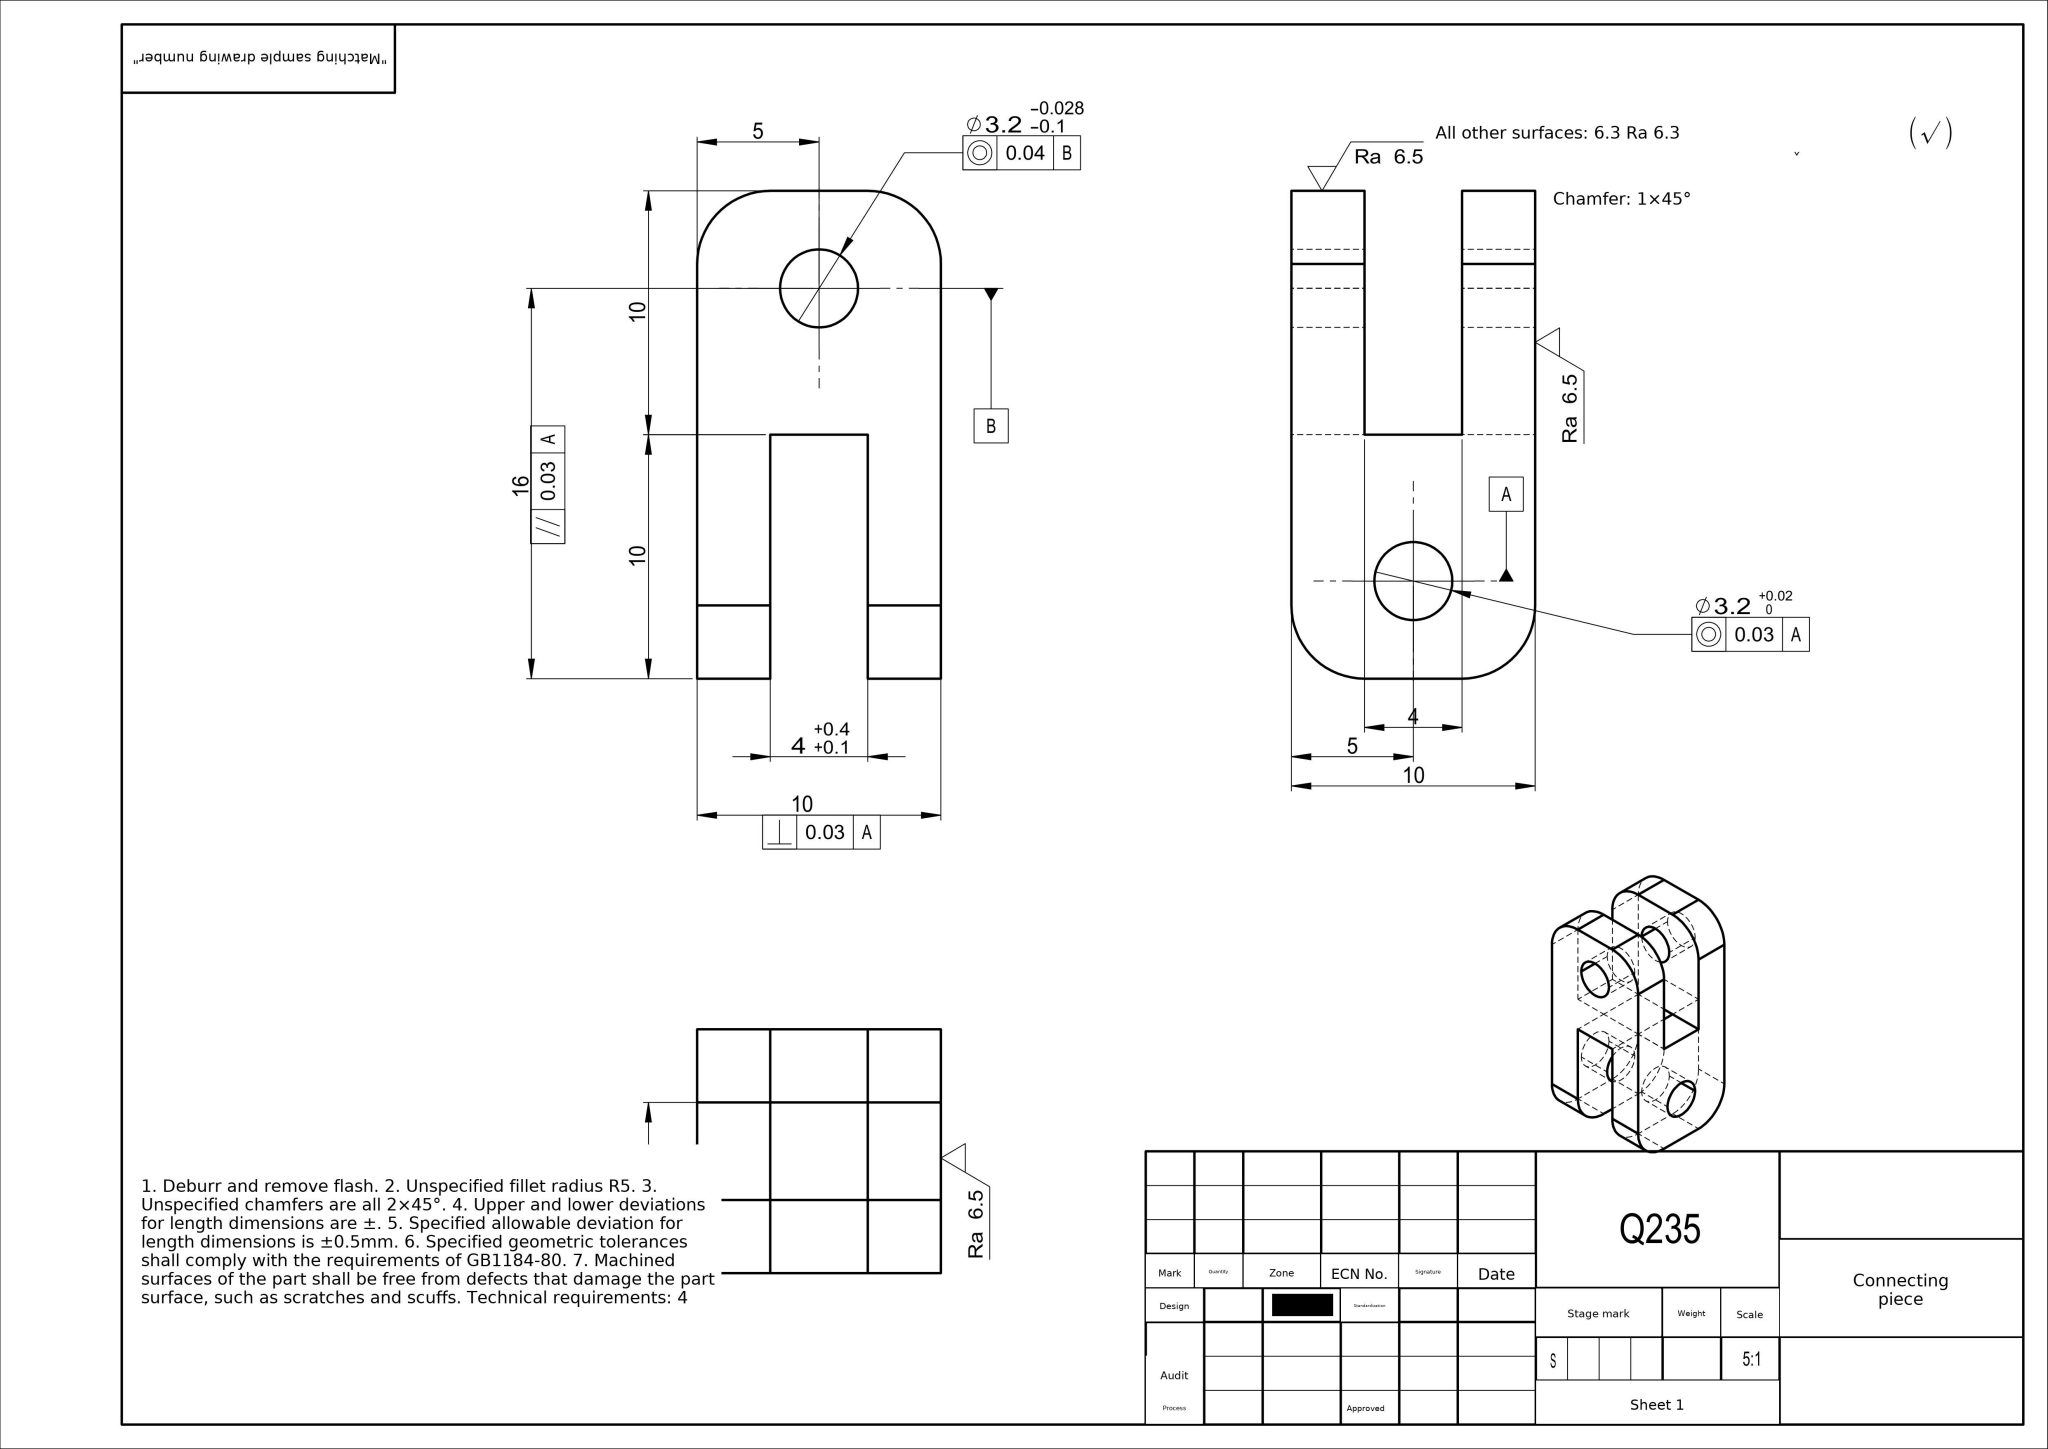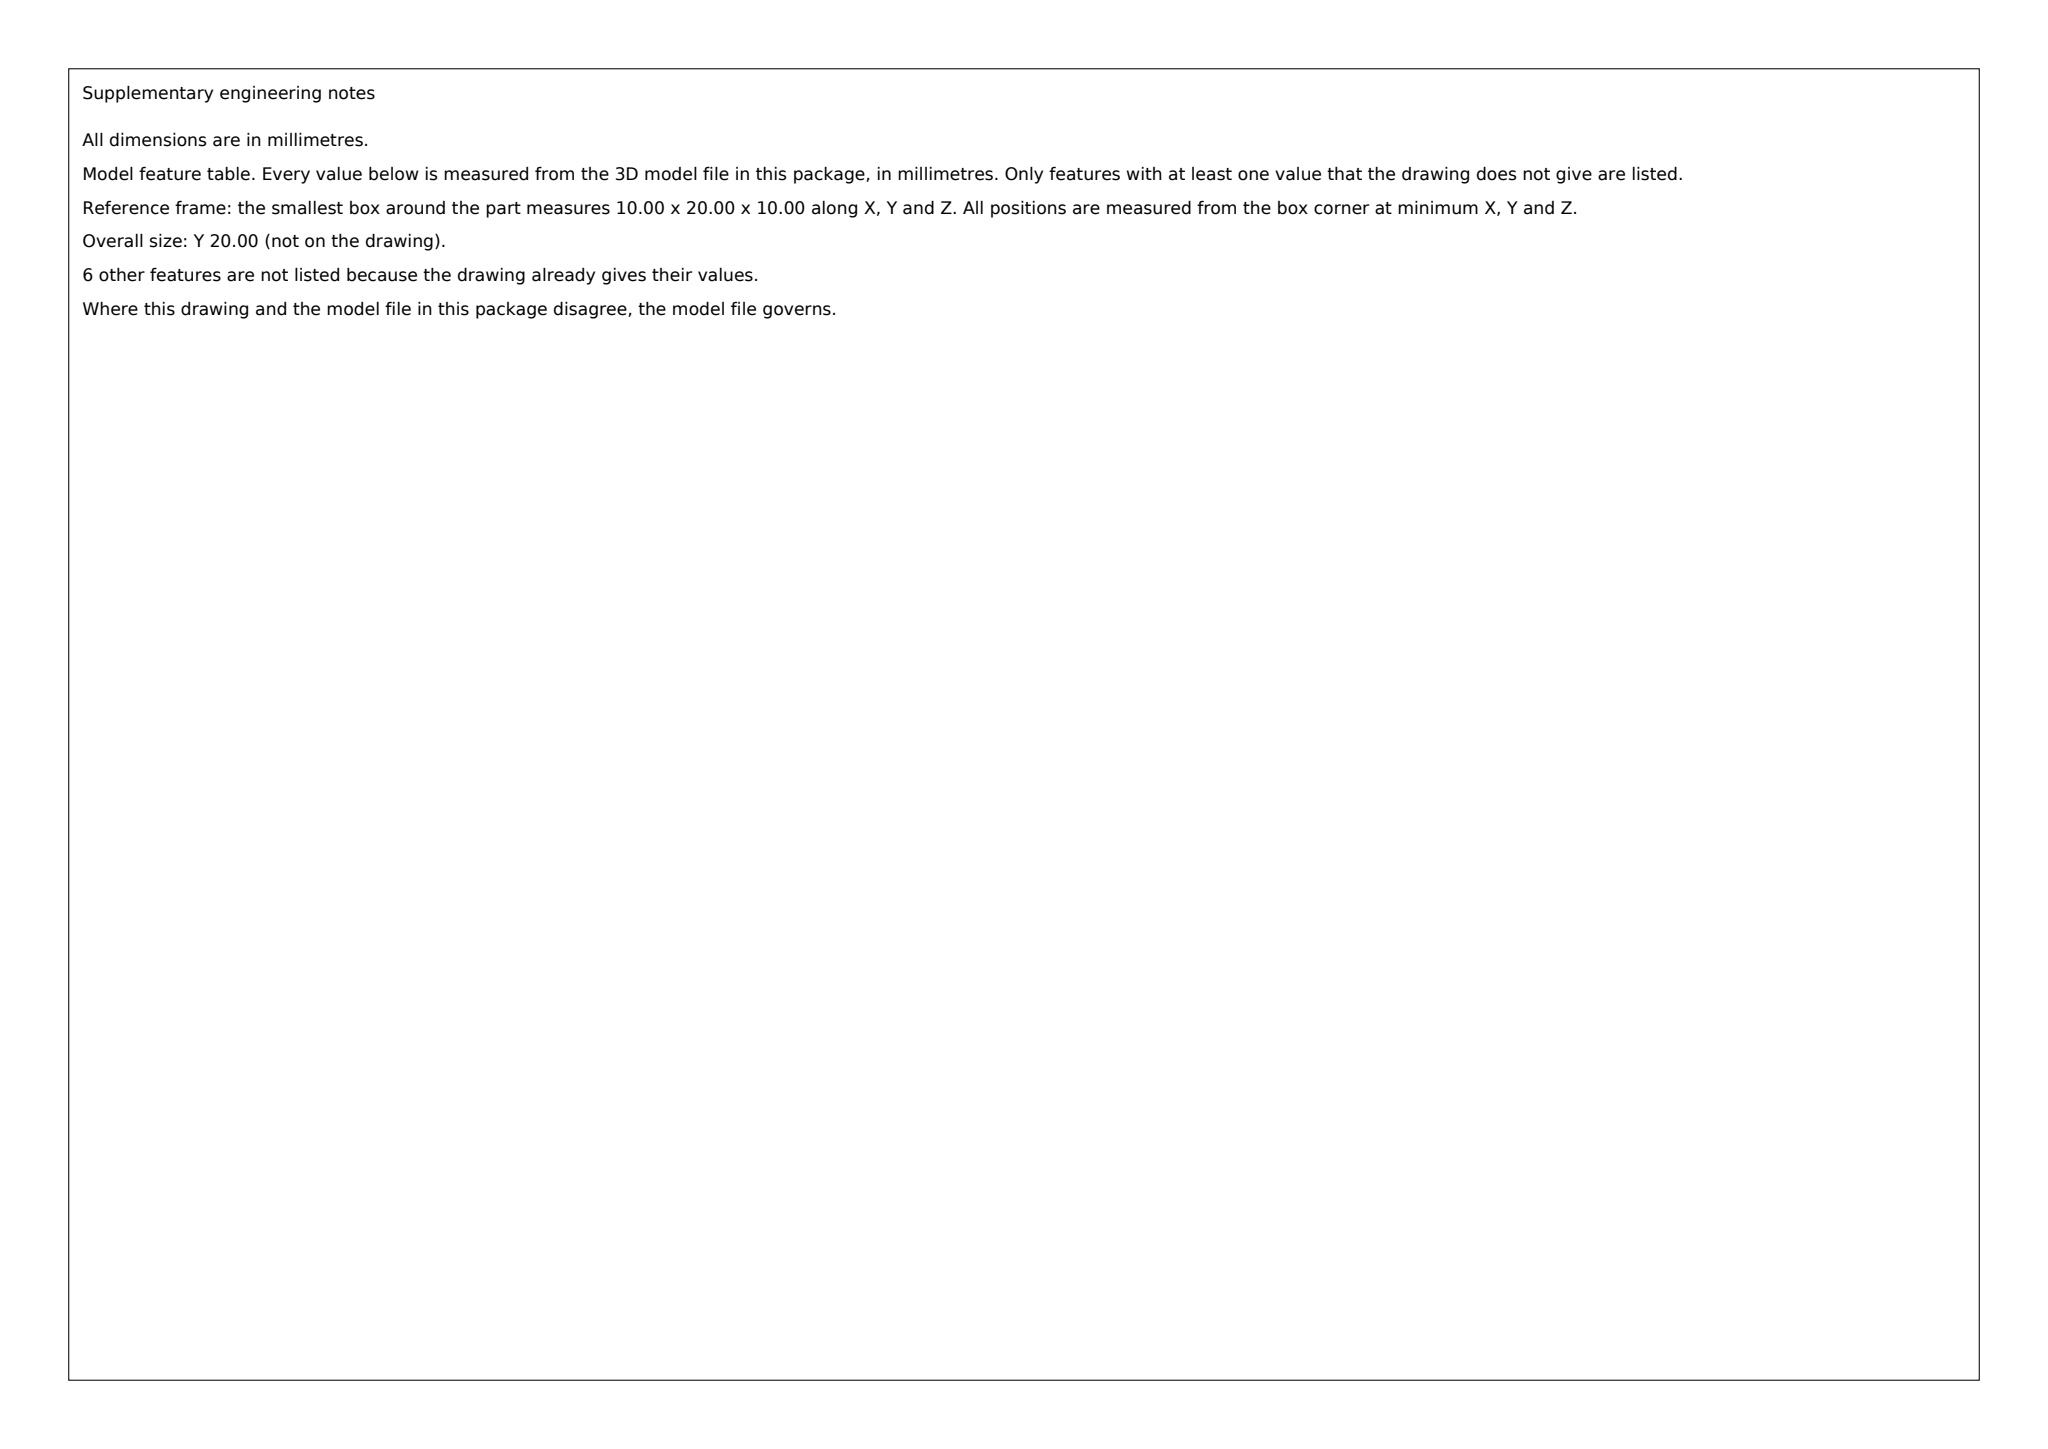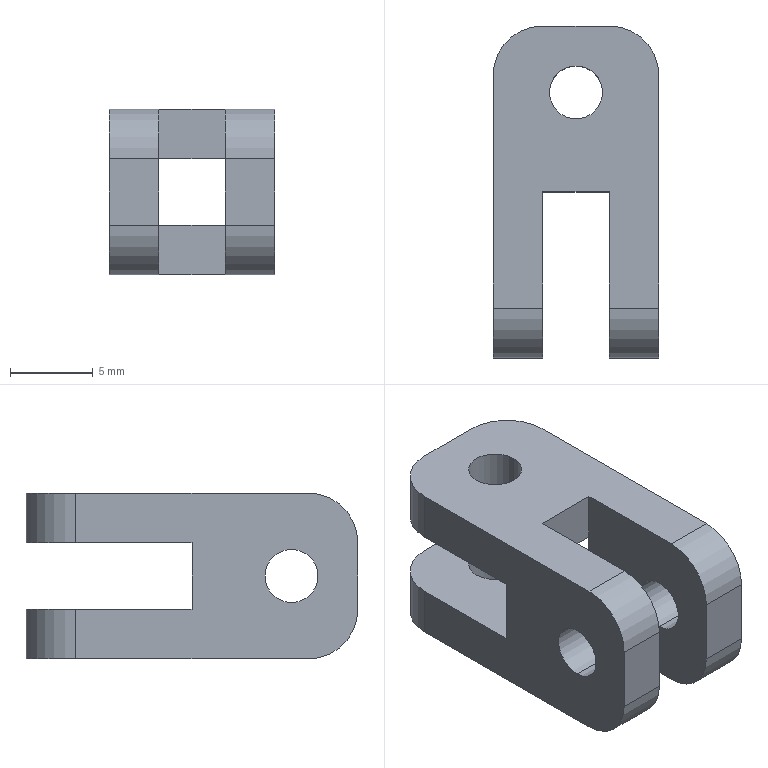Part | SolidWorks | mm | material Q235 | 1 solid | 32 faces | box 10 x 20 x 10 mm | volume 1057 mm3 | cylinder 16 | plane 16 | commonest cylinder face diameters 6 x8 3.2 x8